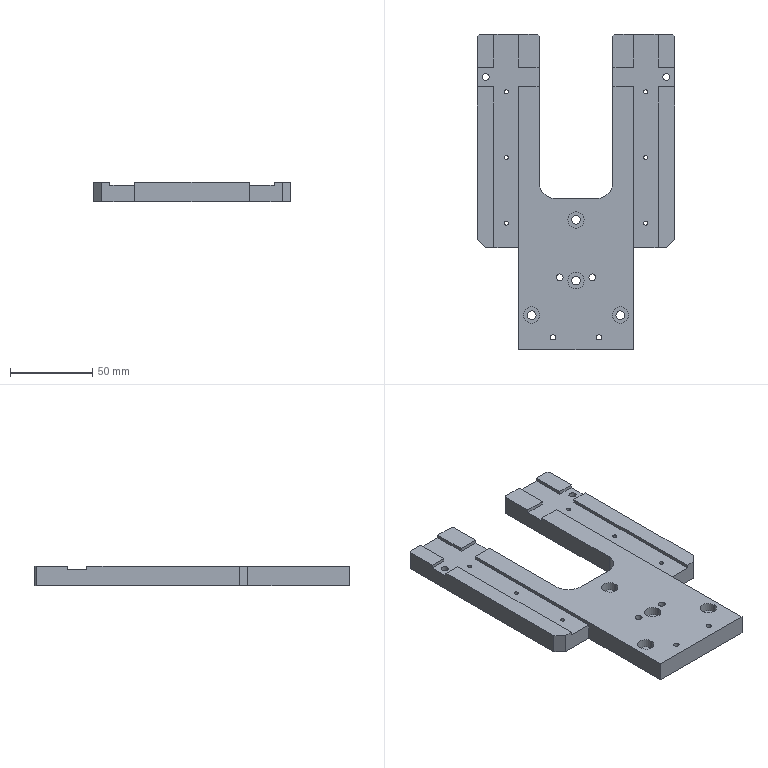Component | SolidWorks | HandlingMechanism-2_A068-1 | 1 solid | 94 faces | box 120 x 192 x 12 mm | volume 172875 mm3 | plane 48 | cylinder 46 | commonest cylinder face diameters 2.5 x12 10 x8 5.3 x8 3.3 x4 8 x4 4.3 x4 4.2 x4 20 x2
build123d program:
from build123d import *

# Parameters (mm, degrees)
SKETCH1_W                                       = 120
SKETCH1_H                                       = 192
BOSS_EXTRUDE1_DEPTH                             = 12
SKETCH3_W                                       = 45
SKETCH3_H                                       = 100
CUT_EXTRUDE2_DEPTH                              = 12
CHAMFER2_SIZE                                   = 1
SKETCH8_W                                       = 25
SKETCH8_H                                       = 62
CUT_EXTRUDE7_DEPTH                              = 20
CHAMFER3_SIZE                                   = 5
SKETCH5_W                                       = 15
SKETCH5_H                                       = 130
CUT_EXTRUDE8_DEPTH                              = 2
SKETCH6_W                                       = 120
SKETCH6_H                                       = 12
CUT_EXTRUDE5_DEPTH                              = 2
M5_TAPPED_HOLE1_D                               = 4.2
M5_TAPPED_HOLE1_DEPTH                           = 14
M5_TAPPED_HOLE1_TIP                             = 1.262
M5_HEX_SOCKET_HEAD_CAP_SCREW_CBORE1_D           = 5.3
M5_HEX_SOCKET_HEAD_CAP_SCREW_CBORE1_CBORE_D     = 10
M5_HEX_SOCKET_HEAD_CAP_SCREW_CBORE1_CBORE_DEPTH = 5.4
M4_HEX_SOCKET_HEAD_CAP_SCREW_CBORE1_D           = 4.3
M4_HEX_SOCKET_HEAD_CAP_SCREW_CBORE1_CBORE_D     = 8
M4_HEX_SOCKET_HEAD_CAP_SCREW_CBORE1_CBORE_DEPTH = 4.4
M4_TAPPED_HOLE1_D                               = 3.3
FILLET1_R                                       = 10
M3_TAPPED_HOLE1_D                               = 2.5


with BuildPart() as part:
    # Sketch1 → Boss-Extrude1 (new body)
    with BuildSketch(Plane.XY):
        Rectangle(SKETCH1_W, SKETCH1_H)
    extrude(amount=BOSS_EXTRUDE1_DEPTH)

    # Sketch3 → Cut-Extrude2 (cut)
    with BuildSketch(Plane.XY.offset(12)):
        with Locations((0, -46)):
            Rectangle(SKETCH3_W, SKETCH3_H)
    extrude(amount=-CUT_EXTRUDE2_DEPTH, mode=Mode.SUBTRACT)

    # Chamfer2
    chamfer2_edges = [part.edges().sort_by_distance(p)[0] for p in [
        (-22.5, -96, 6),
        (22.5, -96, 6),
        (60, -96, 6),
        (-60, -96, 6),
    ]]
    chamfer(chamfer2_edges, length=CHAMFER2_SIZE)

    # Sketch8 → Cut-Extrude7 (cut)
    with BuildSketch(Plane.XY.offset(12)):
        with Locations((-47.5, 65)):
            Rectangle(SKETCH8_W, SKETCH8_H)
        with Locations((47.5, 65)):
            Rectangle(SKETCH8_W, SKETCH8_H)
    extrude(amount=-CUT_EXTRUDE7_DEPTH, mode=Mode.SUBTRACT)

    # Chamfer3
    chamfer3_edges = [part.edges().sort_by_distance(p)[0] for p in [
        (-60, 34, 6),
        (60, 34, 6),
    ]]
    chamfer(chamfer3_edges, length=CHAMFER3_SIZE)

    # Sketch5 → Cut-Extrude8 (cut)
    with BuildSketch(Plane.XY.offset(12)):
        with Locations((-42.5, -31)):
            Rectangle(SKETCH5_W, SKETCH5_H)
        with Locations((42.5, -31)):
            Rectangle(SKETCH5_W, SKETCH5_H)
    extrude(amount=-CUT_EXTRUDE8_DEPTH, mode=Mode.SUBTRACT)

    # Sketch6 → Cut-Extrude5 (cut)
    with BuildSketch(Plane.XY.offset(12)):
        with Locations((0, -70)):
            Rectangle(SKETCH6_W, SKETCH6_H)
    extrude(amount=-CUT_EXTRUDE5_DEPTH, mode=Mode.SUBTRACT)

    # M5 Tapped Hole1
    with Locations(Plane.XY.offset(12)):
        with Locations((-10, 52), (10, 52)):
            Hole(M5_TAPPED_HOLE1_D / 2, depth=M5_TAPPED_HOLE1_DEPTH)
            with Locations((0, 0, -(M5_TAPPED_HOLE1_DEPTH + M5_TAPPED_HOLE1_TIP / 2))):  # 118° drill point
                Cone(0, M5_TAPPED_HOLE1_D / 2, M5_TAPPED_HOLE1_TIP, mode=Mode.SUBTRACT)

    # M5 Hex Socket Head Cap Screw CBORE1 (through all)
    with Locations(Plane(origin=(-11.728, -10.556, 12), x_dir=(-1, 0, 0), z_dir=(0, 0, 1))):
        with Locations((-38.728, -85.556), (15.272, -85.556), (-11.728, -64.556), (-11.728, -27.556)):
            CounterBoreHole(M5_HEX_SOCKET_HEAD_CAP_SCREW_CBORE1_D / 2, M5_HEX_SOCKET_HEAD_CAP_SCREW_CBORE1_CBORE_D / 2, M5_HEX_SOCKET_HEAD_CAP_SCREW_CBORE1_CBORE_DEPTH)

    # M4 Hex Socket Head Cap Screw CBORE1 (through all)
    with Locations(Plane(origin=(0, 0, 0), x_dir=(-1, 0, 0), z_dir=(0, 0, -1))):
        with Locations((55, -70), (-55, -70)):
            CounterBoreHole(M4_HEX_SOCKET_HEAD_CAP_SCREW_CBORE1_D / 2, M4_HEX_SOCKET_HEAD_CAP_SCREW_CBORE1_CBORE_D / 2, M4_HEX_SOCKET_HEAD_CAP_SCREW_CBORE1_CBORE_DEPTH)

    # M4 Tapped Hole1 (through all)
    with Locations(Plane(origin=(0, 0, 0), x_dir=(-1, 0, 0), z_dir=(0, 0, -1))):
        with Locations((14, 88.5), (-14, 88.5)):
            Hole(M4_TAPPED_HOLE1_D / 2)

    # Fillet1
    fillet1_edges = [part.edges().sort_by_distance(p)[0] for p in [
        (-22.5, 4, 6),
        (22.5, 4, 6),
    ]]
    fillet(fillet1_edges, radius=FILLET1_R)

    # M3 Tapped Hole1 (through all)
    with Locations(Plane.XY.offset(10)):
        with Locations((-42.5, 19), (-42.5, -21), (-42.5, -61), (42.5, 19), (42.5, -21), (42.5, -61)):
            Hole(M3_TAPPED_HOLE1_D / 2)


solid = part.part

# Placed as in the assembly
solid = solid.moved(Location((25.881, 120.5, 123), (0, 0, 180)))